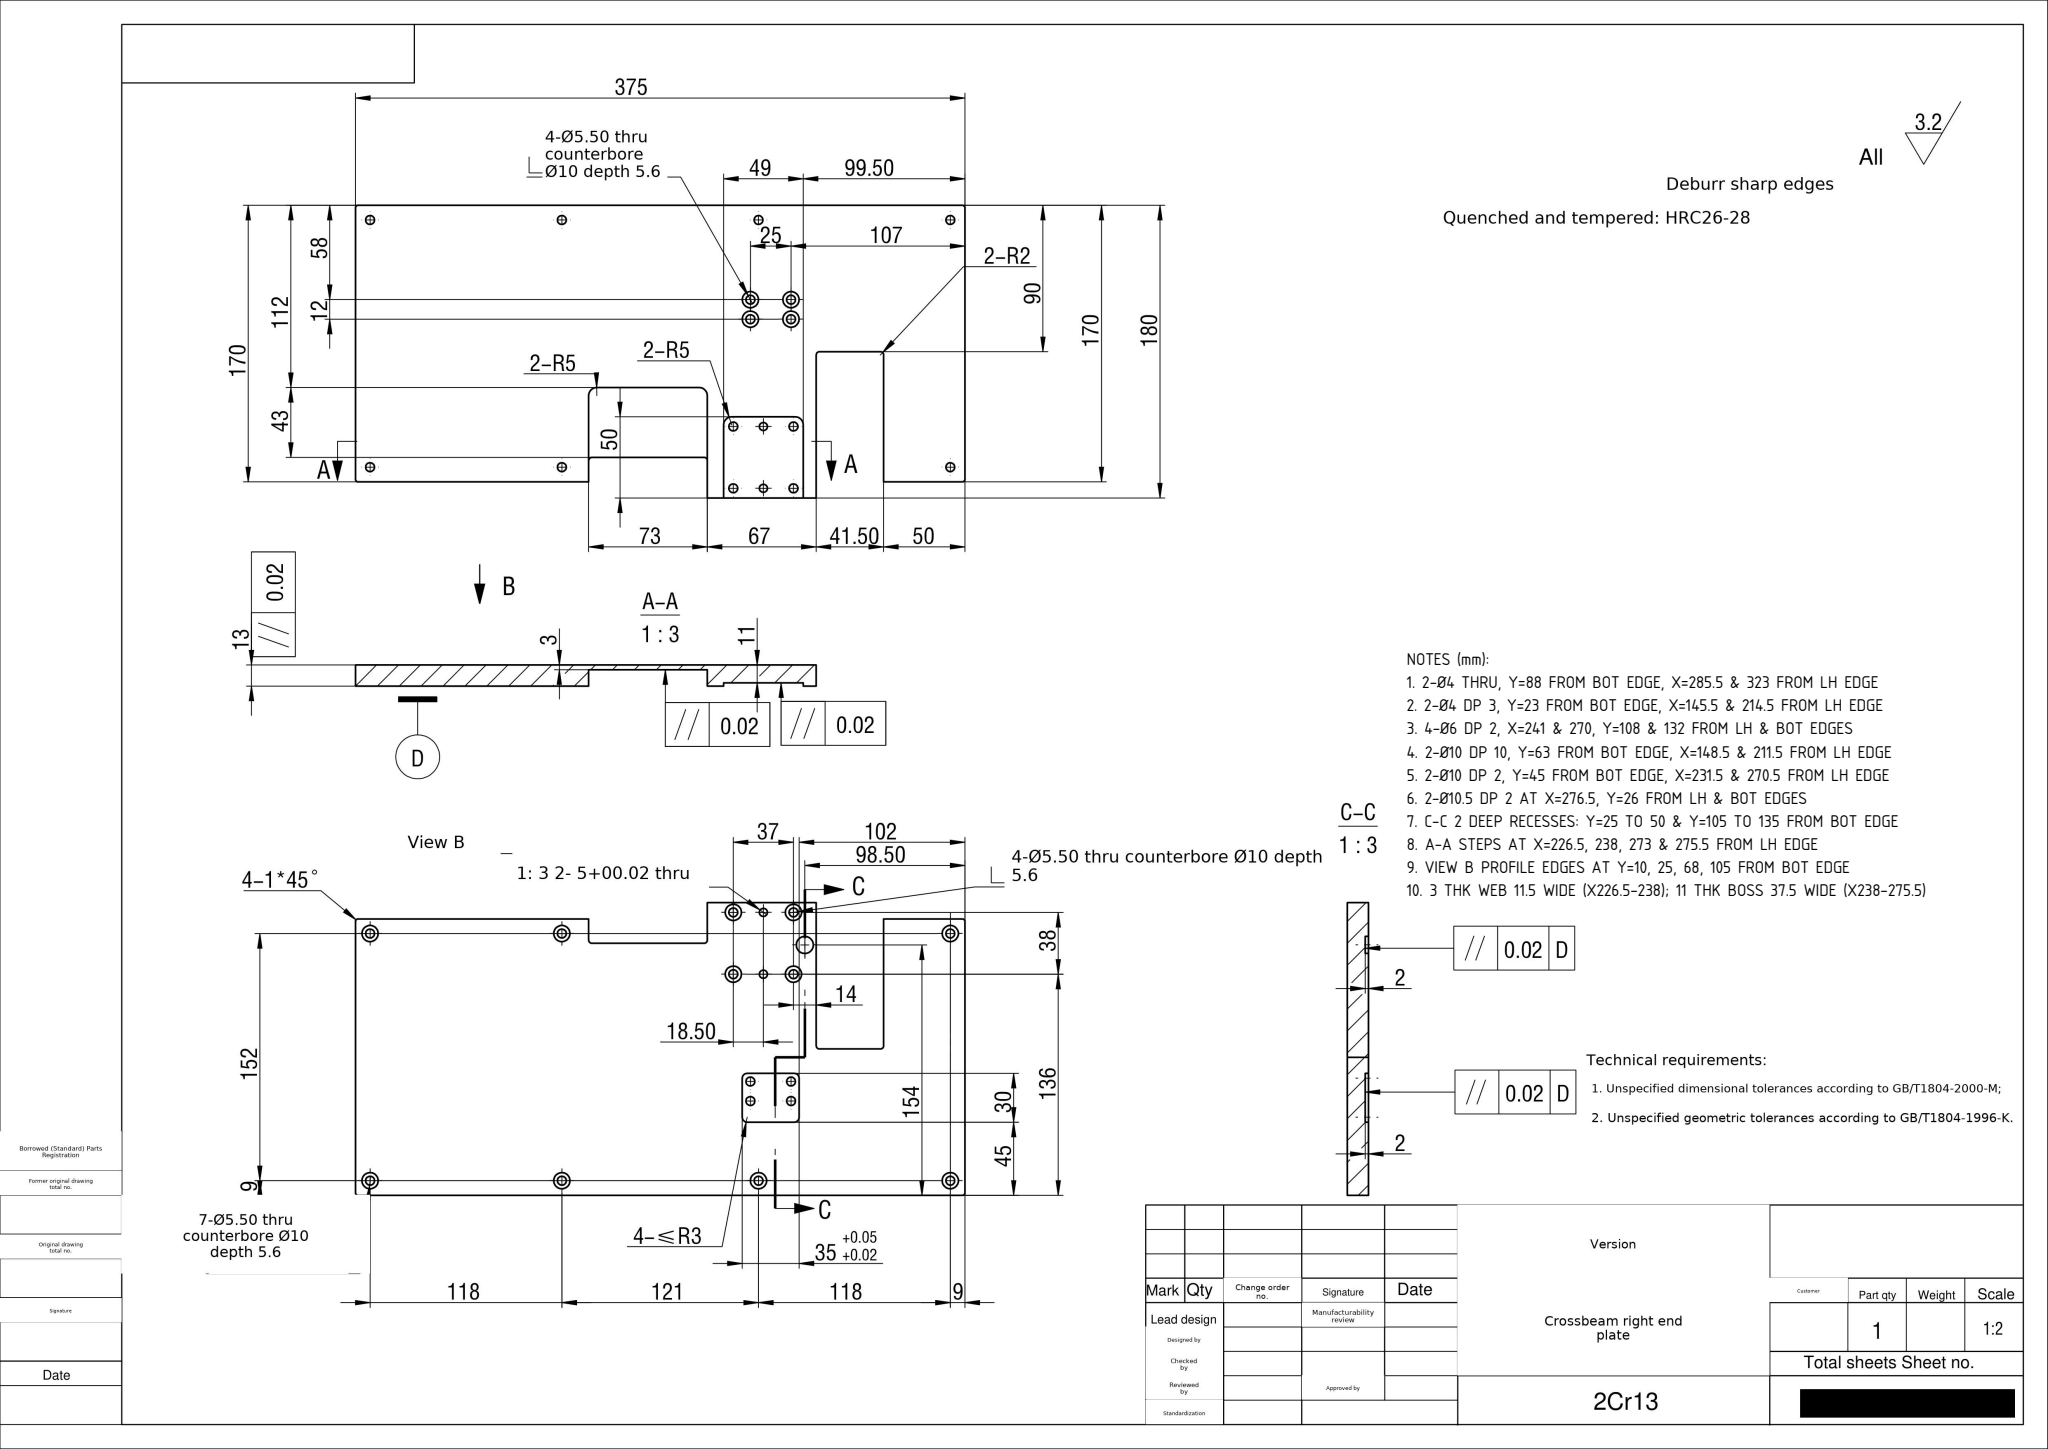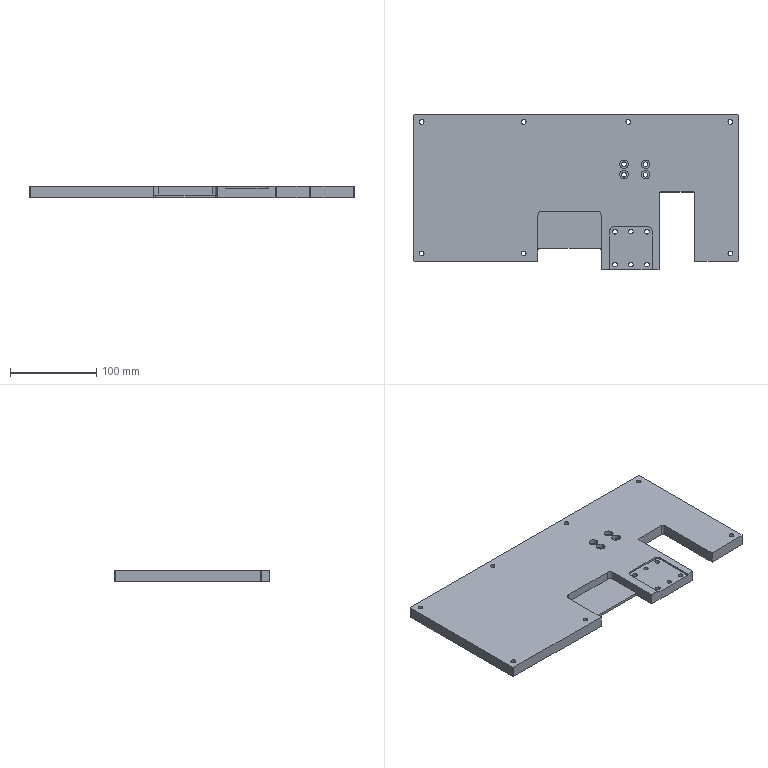Part | SolidWorks | mm | material 2Cr13 | 1 solid | 123 faces | box 375 x 180 x 13 mm | volume 732701 mm3 | cylinder 78 | plane 45 | commonest cylinder face diameters 10 x34 5.5 x30 4 x4 5 x4 6 x4 10.5 x2
Drawing notes:
2-Ø4 THRU, Y=88 FROM BOT EDGE, X=285.5 & 323 FROM LH EDGE | from the solid: cyl Ø4 z-axis at (285.5,88) & (323,88), length 13 = full thk
2-Ø4 DP 3, Y=23 FROM BOT EDGE, X=145.5 & 214.5 FROM LH EDGE | from the solid: cyl Ø4 z-axis at (145.5,23) & (214.5,23), length 3
4-Ø6 DP 2, X=241 & 270, Y=108 & 132 FROM LH & BOT EDGES | from the solid: 4x cyl Ø6 len 2 at (241,108),(241,132),(270,108),(270,132)
2-Ø10 DP 10, Y=63 FROM BOT EDGE, X=148.5 & 211.5 FROM LH EDGE | from the solid: cyl Ø10 len 10 at (148.5,63) & (211.5,63); spacing 63
2-Ø10 DP 2, Y=45 FROM BOT EDGE, X=231.5 & 270.5 FROM LH EDGE | from the solid: cyl Ø10 len 2 at (231.5,45) & (270.5,45)
2-Ø10.5 DP 2 AT X=276.5, Y=26 FROM LH & BOT EDGES | from the solid: cyl Ø10.5 len 2 at (276.5,26), count 2
C-C 2 DEEP RECESSES: Y=25 TO 50 & Y=105 TO 135 FROM BOT EDGE | from the solid: z=2 planes (count 2); y planes 25/50 and 105/135 bound them
A-A STEPS AT X=226.5, 238, 273 & 275.5 FROM LH EDGE | from the solid: x-normal planes at 226.5, 238, 273, 275.5
VIEW B PROFILE EDGES AT Y=10, 25, 68, 105 FROM BOT EDGE | from the solid: y-normal planes at 10, 25, 68, 105
3 THK WEB 11.5 WIDE (X226.5-238); 11 THK BOSS 37.5 WIDE (X238-275.5) | from the solid: z=3 and z=11 regions bounded by x planes 226.5/238/275.5